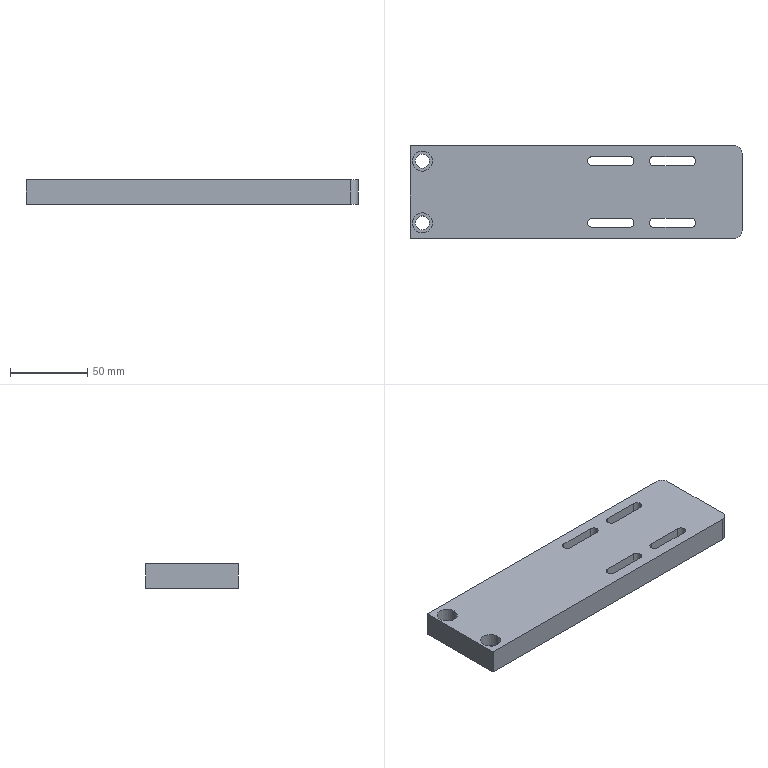CAM job | Mastercam | mm | 12 operations | part box 215 x 60 x 16
1. Facing | 24 - 100 平铣刀
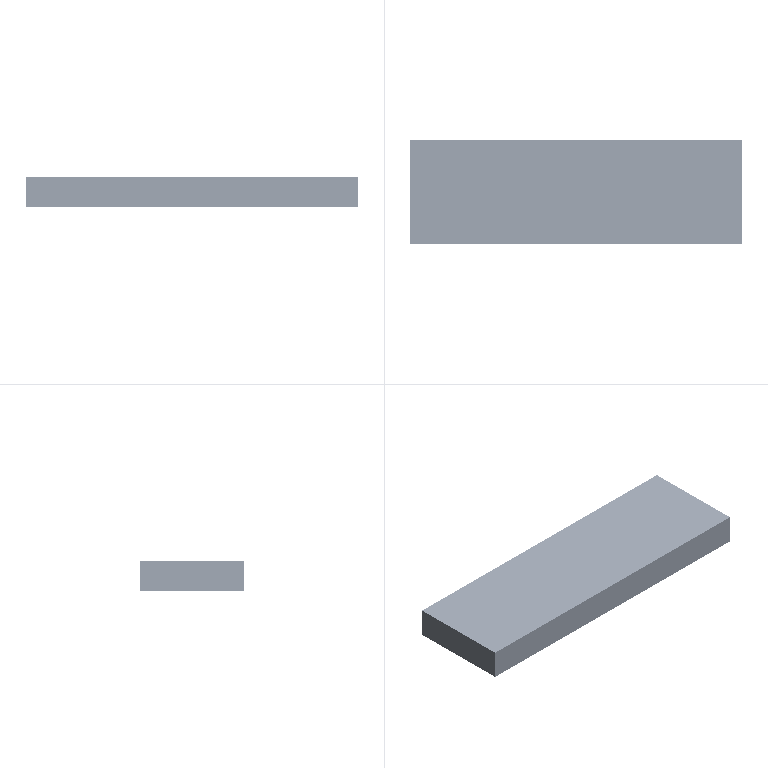2. 2D High Speed (2D Dynamic Mill) | 10 - 10 平铣刀
3. Drill/Counterbore | 7 - 6 倒角刀
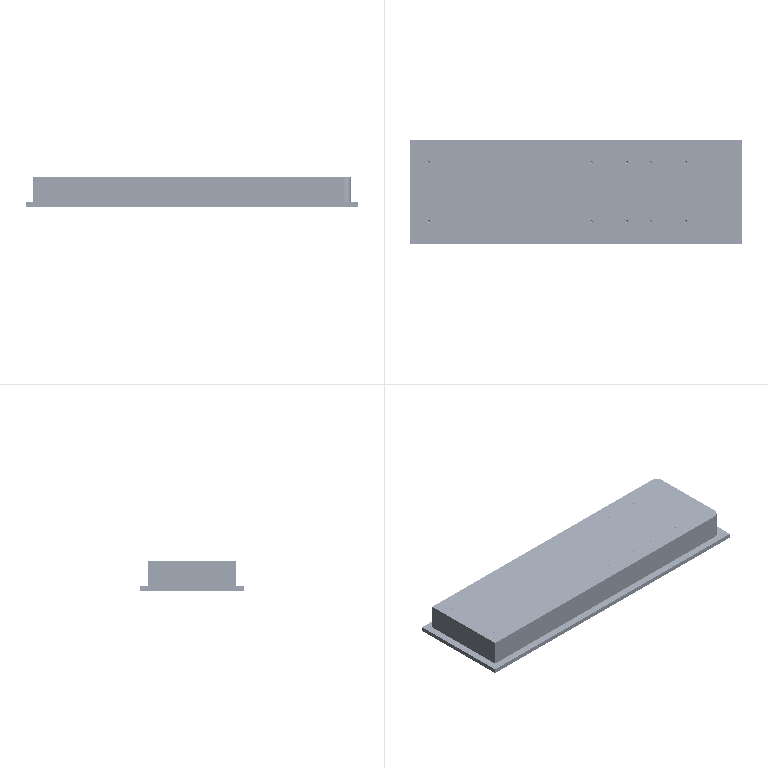4. Peck Drill | 1 - 5.5 钻头
5. Helix Bore | 6 - 6 平铣刀
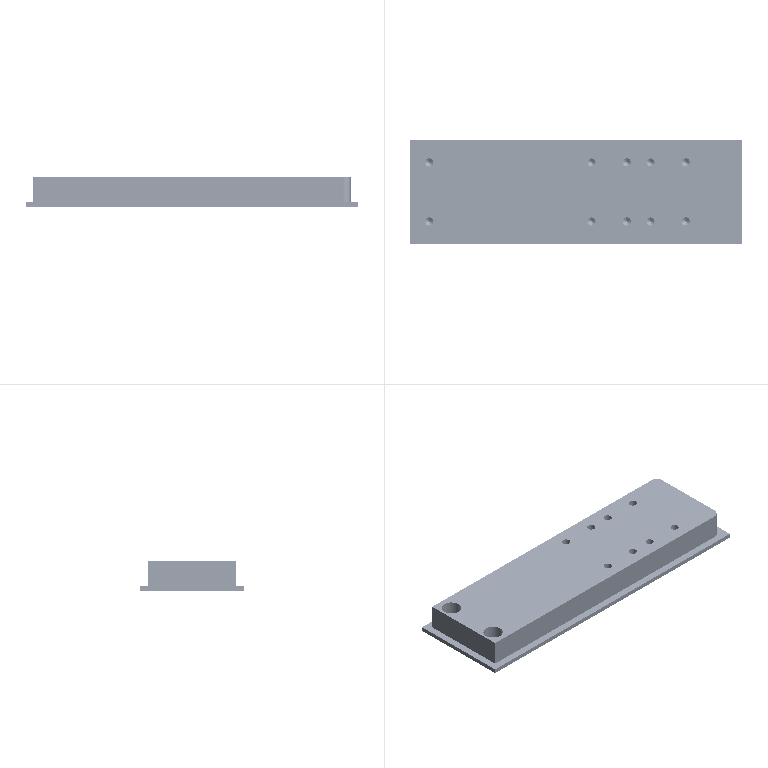6. Contour (Ramp) | 5 - 5 平铣刀
7. Helix Bore | 5 - 5 平铣刀
8. Contour (Ramp) | 5 - 5 平铣刀
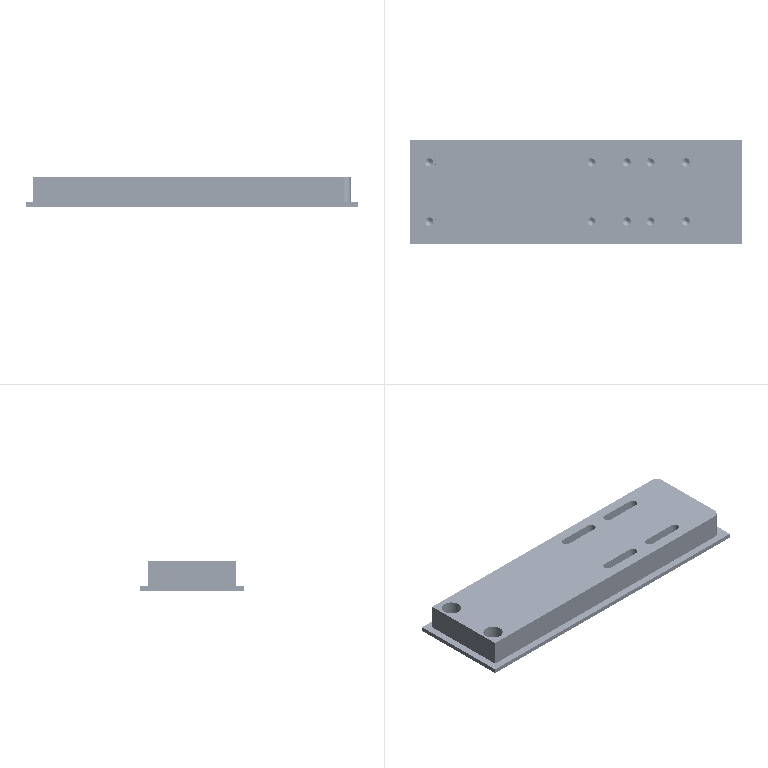9. Contour (2D) | 21 - 12 平铣刀
10. Model Chamfer | 7 - 6 倒角刀
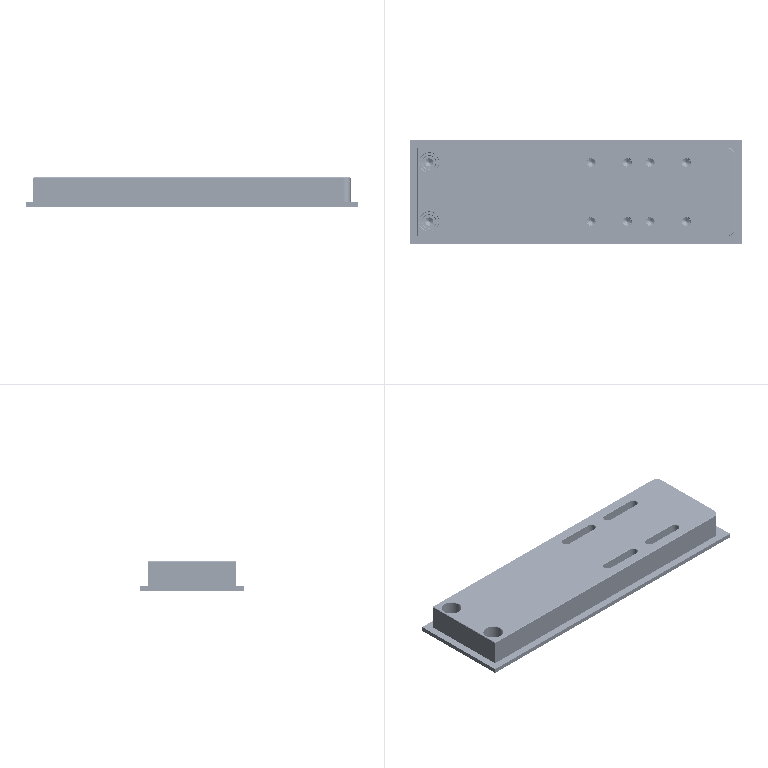11. Facing | 24 - 100 平铣刀
12. Contour (2D chamfer) | 7 - 6 倒角刀